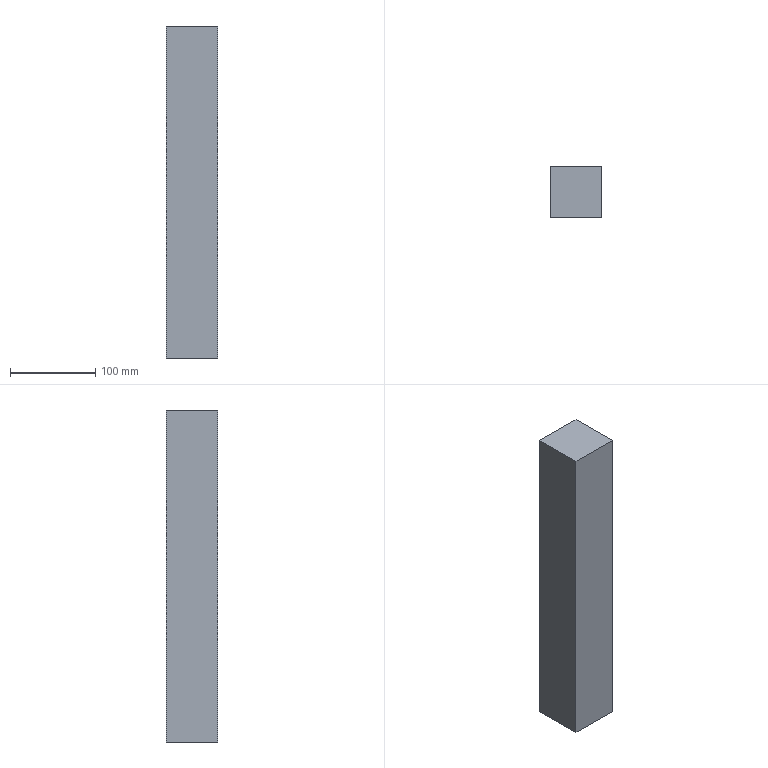Component | SolidWorks | JF21-80.1-1-3(_)-1-SOLID60-1 | 1 solid | 6 faces | box 60 x 60 x 390 mm | volume 1404000 mm3 | plane 6
STEP:
#1=COLOUR_RGB('',0.7922,0.8196,0.9333);
#2=FILL_AREA_STYLE_COLOUR('',#1);
#3=FILL_AREA_STYLE('',(#2));
#4=SURFACE_STYLE_FILL_AREA(#3);
#5=SURFACE_SIDE_STYLE('',(#4));
#6=SURFACE_STYLE_USAGE(.BOTH.,#5);
#7=PRESENTATION_STYLE_ASSIGNMENT((#6));
#8=CARTESIAN_POINT('',(12.598,-62.205,7.677));
#9=VERTEX_POINT('',#8);
#10=CARTESIAN_POINT('',(12.598,-62.205,-7.677));
#11=VERTEX_POINT('',#10);
#12=CARTESIAN_POINT('',(12.598,-62.205,-7.677));
#13=DIRECTION('',(0.,0.,-1.));
#14=VECTOR('',#13,39.37);
#15=LINE('',#12,#14);
#16=EDGE_CURVE('',#9,#11,#15,.T.);
#17=ORIENTED_EDGE('',*,*,#16,.F.);
#18=CARTESIAN_POINT('',(12.598,-64.567,7.677));
#19=VERTEX_POINT('',#18);
#20=CARTESIAN_POINT('',(12.598,-64.567,7.677));
#21=DIRECTION('',(0.,1.,0.));
#22=VECTOR('',#21,39.37);
#23=LINE('',#20,#22);
#24=EDGE_CURVE('',#19,#9,#23,.T.);
#25=ORIENTED_EDGE('',*,*,#24,.F.);
#26=CARTESIAN_POINT('',(12.598,-64.567,-7.677));
#27=VERTEX_POINT('',#26);
#28=CARTESIAN_POINT('',(12.598,-64.567,-7.677));
#29=DIRECTION('',(0.,0.,-1.));
#30=VECTOR('',#29,39.37);
#31=LINE('',#28,#30);
#32=EDGE_CURVE('',#19,#27,#31,.T.);
#33=ORIENTED_EDGE('',*,*,#32,.T.);
#34=CARTESIAN_POINT('',(12.598,-64.567,-7.677));
#35=DIRECTION('',(0.,1.,0.));
#36=VECTOR('',#35,39.37);
#37=LINE('',#34,#36);
#38=EDGE_CURVE('',#27,#11,#37,.T.);
#39=ORIENTED_EDGE('',*,*,#38,.T.);
#40=EDGE_LOOP('',(#17,#25,#33,#39));
#41=FACE_OUTER_BOUND('',#40,.T.);
#42=CARTESIAN_POINT('',(12.598,-64.567,-7.677));
#43=DIRECTION('',(1.,0.,0.));
#44=DIRECTION('',(0.,0.,1.));
#45=AXIS2_PLACEMENT_3D('',#42,#43,#44);
#46=PLANE('',#45);
#47=ADVANCED_FACE('',(#41),#46,.T.);
#48=CARTESIAN_POINT('',(10.236,-62.205,7.677));
#49=VERTEX_POINT('',#48);
#50=CARTESIAN_POINT('',(12.598,-62.205,7.677));
#51=DIRECTION('',(1.,0.,0.));
#52=VECTOR('',#51,39.37);
#53=LINE('',#50,#52);
#54=EDGE_CURVE('',#49,#9,#53,.T.);
#55=ORIENTED_EDGE('',*,*,#54,.F.);
#56=CARTESIAN_POINT('',(10.236,-64.567,7.677));
#57=VERTEX_POINT('',#56);
#58=CARTESIAN_POINT('',(10.236,-64.567,7.677));
#59=DIRECTION('',(0.,1.,0.));
#60=VECTOR('',#59,39.37);
#61=LINE('',#58,#60);
#62=EDGE_CURVE('',#57,#49,#61,.T.);
#63=ORIENTED_EDGE('',*,*,#62,.F.);
#64=CARTESIAN_POINT('',(12.598,-64.567,7.677));
#65=DIRECTION('',(1.,0.,0.));
#66=VECTOR('',#65,39.37);
#67=LINE('',#64,#66);
#68=EDGE_CURVE('',#57,#19,#67,.T.);
#69=ORIENTED_EDGE('',*,*,#68,.T.);
#70=ORIENTED_EDGE('',*,*,#24,.T.);
#71=EDGE_LOOP('',(#55,#63,#69,#70));
#72=FACE_OUTER_BOUND('',#71,.T.);
#73=CARTESIAN_POINT('',(12.598,-64.567,7.677));
#74=DIRECTION('',(0.,0.,1.));
#75=DIRECTION('',(-1.,0.,0.));
#76=AXIS2_PLACEMENT_3D('',#73,#74,#75);
#77=PLANE('',#76);
#78=ADVANCED_FACE('',(#72),#77,.T.);
#79=CARTESIAN_POINT('',(10.236,-62.205,-7.677));
#80=VERTEX_POINT('',#79);
#81=CARTESIAN_POINT('',(10.236,-62.205,-7.677));
#82=DIRECTION('',(0.,0.,1.));
#83=VECTOR('',#82,39.37);
#84=LINE('',#81,#83);
#85=EDGE_CURVE('',#80,#49,#84,.T.);
#86=ORIENTED_EDGE('',*,*,#85,.F.);
#87=CARTESIAN_POINT('',(10.236,-64.567,-7.677));
#88=VERTEX_POINT('',#87);
#89=CARTESIAN_POINT('',(10.236,-64.567,-7.677));
#90=DIRECTION('',(0.,1.,0.));
#91=VECTOR('',#90,39.37);
#92=LINE('',#89,#91);
#93=EDGE_CURVE('',#88,#80,#92,.T.);
#94=ORIENTED_EDGE('',*,*,#93,.F.);
#95=CARTESIAN_POINT('',(10.236,-64.567,-7.677));
#96=DIRECTION('',(0.,0.,1.));
#97=VECTOR('',#96,39.37);
#98=LINE('',#95,#97);
#99=EDGE_CURVE('',#88,#57,#98,.T.);
#100=ORIENTED_EDGE('',*,*,#99,.T.);
#101=ORIENTED_EDGE('',*,*,#62,.T.);
#102=EDGE_LOOP('',(#86,#94,#100,#101));
#103=FACE_OUTER_BOUND('',#102,.T.);
#104=CARTESIAN_POINT('',(10.236,-64.567,-7.677));
#105=DIRECTION('',(-1.,0.,0.));
#106=DIRECTION('',(-0.,0.,-1.));
#107=AXIS2_PLACEMENT_3D('',#104,#105,#106);
#108=PLANE('',#107);
#109=ADVANCED_FACE('',(#103),#108,.T.);
#110=CARTESIAN_POINT('',(12.598,-62.205,-7.677));
#111=DIRECTION('',(-1.,0.,0.));
#112=VECTOR('',#111,39.37);
#113=LINE('',#110,#112);
#114=EDGE_CURVE('',#11,#80,#113,.T.);
#115=ORIENTED_EDGE('',*,*,#114,.F.);
#116=ORIENTED_EDGE('',*,*,#38,.F.);
#117=CARTESIAN_POINT('',(12.598,-64.567,-7.677));
#118=DIRECTION('',(-1.,0.,0.));
#119=VECTOR('',#118,39.37);
#120=LINE('',#117,#119);
#121=EDGE_CURVE('',#27,#88,#120,.T.);
#122=ORIENTED_EDGE('',*,*,#121,.T.);
#123=ORIENTED_EDGE('',*,*,#93,.T.);
#124=EDGE_LOOP('',(#115,#116,#122,#123));
#125=FACE_OUTER_BOUND('',#124,.T.);
#126=CARTESIAN_POINT('',(12.598,-64.567,-7.677));
#127=DIRECTION('',(-0.,0.,-1.));
#128=DIRECTION('',(1.,0.,-0.));
#129=AXIS2_PLACEMENT_3D('',#126,#127,#128);
#130=PLANE('',#129);
#131=ADVANCED_FACE('',(#125),#130,.T.);
#132=ORIENTED_EDGE('',*,*,#32,.F.);
#133=ORIENTED_EDGE('',*,*,#68,.F.);
#134=ORIENTED_EDGE('',*,*,#99,.F.);
#135=ORIENTED_EDGE('',*,*,#121,.F.);
#136=EDGE_LOOP('',(#132,#133,#134,#135));
#137=FACE_OUTER_BOUND('',#136,.T.);
#138=CARTESIAN_POINT('',(12.598,-64.567,7.677));
#139=DIRECTION('',(0.,-1.,0.));
#140=DIRECTION('',(0.,0.,1.));
#141=AXIS2_PLACEMENT_3D('',#138,#139,#140);
#142=PLANE('',#141);
#143=ADVANCED_FACE('',(#137),#142,.T.);
#144=ORIENTED_EDGE('',*,*,#16,.T.);
#145=ORIENTED_EDGE('',*,*,#114,.T.);
#146=ORIENTED_EDGE('',*,*,#85,.T.);
#147=ORIENTED_EDGE('',*,*,#54,.T.);
#148=EDGE_LOOP('',(#144,#145,#146,#147));
#149=FACE_OUTER_BOUND('',#148,.T.);
#150=CARTESIAN_POINT('',(12.598,-62.205,7.677));
#151=DIRECTION('',(0.,-1.,0.));
#152=DIRECTION('',(0.,0.,1.));
#153=AXIS2_PLACEMENT_3D('',#150,#151,#152);
#154=PLANE('',#153);
#155=ADVANCED_FACE('',(#149),#154,.F.);
#156=CLOSED_SHELL('',(#47,#78,#109,#131,#143,#155));
#157=MANIFOLD_SOLID_BREP('',#156);
#158=STYLED_ITEM('',(#7),#157);
#159=PRESENTATION_LAYER_ASSIGNMENT('','',(#158));
#160=(LENGTH_UNIT()NAMED_UNIT(*)SI_UNIT($,.METRE.));
#161=LENGTH_MEASURE_WITH_UNIT(LENGTH_MEASURE(0.0254),#160);
#162=DIMENSIONAL_EXPONENTS(1.,0.,0.,0.,0.,0.,0.);
#163=(CONVERSION_BASED_UNIT('',#161)LENGTH_UNIT()NAMED_UNIT(#162));
#164=UNCERTAINTY_MEASURE_WITH_UNIT(LENGTH_MEASURE(0.00001),#163,'','');
#165=(NAMED_UNIT(*)PLANE_ANGLE_UNIT()SI_UNIT($,.RADIAN.));
#166=(NAMED_UNIT(*)SI_UNIT($,.STERADIAN.)SOLID_ANGLE_UNIT());
#167=(GEOMETRIC_REPRESENTATION_CONTEXT(3)GLOBAL_UNCERTAINTY_ASSIGNED_CONTEXT((#164))GLOBAL_UNIT_ASSIGNED_CONTEXT((#163,#165,#166))REPRESENTATION_CONTEXT('',''));
#168=MECHANICAL_DESIGN_GEOMETRIC_PRESENTATION_REPRESENTATION('',(#158),#167);
#169=CARTESIAN_POINT('',(0.,0.,0.));
#170=DIRECTION('',(0.,0.,1.));
#171=DIRECTION('',(1.,0.,0.));
#172=AXIS2_PLACEMENT_3D('',#169,#170,#171);
#173=(LENGTH_UNIT()NAMED_UNIT(*)SI_UNIT($,.METRE.));
#174=LENGTH_MEASURE_WITH_UNIT(LENGTH_MEASURE(0.0254),#173);
#175=DIMENSIONAL_EXPONENTS(1.,0.,0.,0.,0.,0.,0.);
#176=(CONVERSION_BASED_UNIT('',#174)LENGTH_UNIT()NAMED_UNIT(#175));
#177=UNCERTAINTY_MEASURE_WITH_UNIT(LENGTH_MEASURE(0.00001),#176,'','');
#178=(NAMED_UNIT(*)PLANE_ANGLE_UNIT()SI_UNIT($,.RADIAN.));
#179=(NAMED_UNIT(*)SI_UNIT($,.STERADIAN.)SOLID_ANGLE_UNIT());
#180=(GEOMETRIC_REPRESENTATION_CONTEXT(3)GLOBAL_UNCERTAINTY_ASSIGNED_CONTEXT((#177))GLOBAL_UNIT_ASSIGNED_CONTEXT((#176,#178,#179))REPRESENTATION_CONTEXT('',''));
#181=ADVANCED_BREP_SHAPE_REPRESENTATION('',(#157,#172),#180);